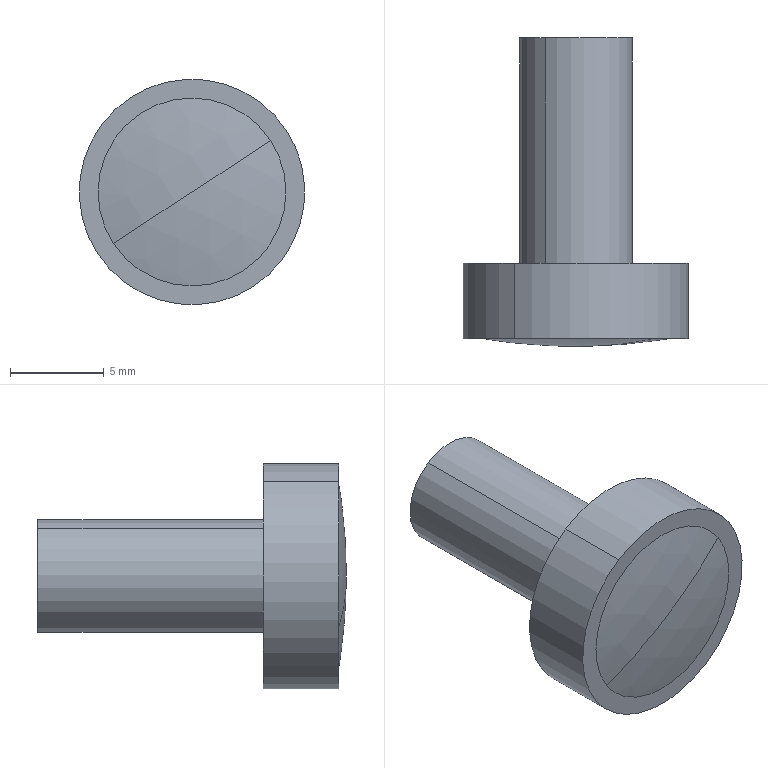Component | SolidWorks | SmallHandwheel-2 | 1 solid | 9 faces | box 12 x 16.42 x 12 mm | volume 808 mm3 | cylinder 4 | plane 3 | sphere 2 | commonest cylinder face diameters 6 x2 12 x2
STEP:
#1=CARTESIAN_POINT('',(7.97,20.827,-9.056));
#2=VERTEX_POINT('',#1);
#3=CARTESIAN_POINT('',(7.841,20.827,-8.858));
#4=VERTEX_POINT('',#3);
#5=CARTESIAN_POINT('',(7.905,20.827,-8.957));
#6=DIRECTION('',(0.,1.,-0.));
#7=DIRECTION('',(0.5469,0.,-0.8372));
#8=AXIS2_PLACEMENT_3D('',#5,#6,#7);
#9=CIRCLE('',#8,0.1181);
#10=EDGE_CURVE('',#2,#4,#9,.T.);
#11=ORIENTED_EDGE('',*,*,#10,.T.);
#12=CARTESIAN_POINT('',(7.841,21.299,-8.858));
#13=VERTEX_POINT('',#12);
#14=CARTESIAN_POINT('',(7.841,21.299,-8.858));
#15=DIRECTION('',(0.,1.,-0.));
#16=VECTOR('',#15,39.37);
#17=LINE('',#14,#16);
#18=EDGE_CURVE('',#4,#13,#17,.T.);
#19=ORIENTED_EDGE('',*,*,#18,.T.);
#20=CARTESIAN_POINT('',(7.97,21.299,-9.056));
#21=VERTEX_POINT('',#20);
#22=CARTESIAN_POINT('',(7.905,21.299,-8.957));
#23=DIRECTION('',(-0.,-1.,0.));
#24=DIRECTION('',(0.5469,0.,-0.8372));
#25=AXIS2_PLACEMENT_3D('',#22,#23,#24);
#26=CIRCLE('',#25,0.1181);
#27=EDGE_CURVE('',#13,#21,#26,.T.);
#28=ORIENTED_EDGE('',*,*,#27,.T.);
#29=CARTESIAN_POINT('',(7.97,21.299,-9.056));
#30=DIRECTION('',(0.,1.,-0.));
#31=VECTOR('',#30,39.37);
#32=LINE('',#29,#31);
#33=EDGE_CURVE('',#2,#21,#32,.T.);
#34=ORIENTED_EDGE('',*,*,#33,.F.);
#35=EDGE_LOOP('',(#11,#19,#28,#34));
#36=FACE_OUTER_BOUND('',#35,.T.);
#37=CARTESIAN_POINT('',(7.905,21.299,-8.957));
#38=DIRECTION('',(0.,1.,-0.));
#39=DIRECTION('',(0.5469,0.,-0.8372));
#40=AXIS2_PLACEMENT_3D('',#37,#38,#39);
#41=CYLINDRICAL_SURFACE('',#40,0.1181);
#42=ADVANCED_FACE('',(#36),#41,.T.);
#43=CARTESIAN_POINT('',(8.034,20.669,-9.154));
#44=VERTEX_POINT('',#43);
#45=CARTESIAN_POINT('',(7.776,20.669,-8.759));
#46=VERTEX_POINT('',#45);
#47=CARTESIAN_POINT('',(7.905,20.669,-8.957));
#48=DIRECTION('',(0.,1.,-0.));
#49=DIRECTION('',(0.5469,0.,-0.8372));
#50=AXIS2_PLACEMENT_3D('',#47,#48,#49);
#51=CIRCLE('',#50,0.2362);
#52=EDGE_CURVE('',#44,#46,#51,.T.);
#53=ORIENTED_EDGE('',*,*,#52,.T.);
#54=CARTESIAN_POINT('',(7.776,20.827,-8.759));
#55=VERTEX_POINT('',#54);
#56=CARTESIAN_POINT('',(7.776,21.299,-8.759));
#57=DIRECTION('',(0.,1.,-0.));
#58=VECTOR('',#57,39.37);
#59=LINE('',#56,#58);
#60=EDGE_CURVE('',#46,#55,#59,.T.);
#61=ORIENTED_EDGE('',*,*,#60,.T.);
#62=CARTESIAN_POINT('',(8.034,20.827,-9.154));
#63=VERTEX_POINT('',#62);
#64=CARTESIAN_POINT('',(7.905,20.827,-8.957));
#65=DIRECTION('',(-0.,-1.,0.));
#66=DIRECTION('',(0.5469,0.,-0.8372));
#67=AXIS2_PLACEMENT_3D('',#64,#65,#66);
#68=CIRCLE('',#67,0.2362);
#69=EDGE_CURVE('',#55,#63,#68,.T.);
#70=ORIENTED_EDGE('',*,*,#69,.T.);
#71=CARTESIAN_POINT('',(8.034,21.299,-9.154));
#72=DIRECTION('',(0.,1.,-0.));
#73=VECTOR('',#72,39.37);
#74=LINE('',#71,#73);
#75=EDGE_CURVE('',#44,#63,#74,.T.);
#76=ORIENTED_EDGE('',*,*,#75,.F.);
#77=EDGE_LOOP('',(#53,#61,#70,#76));
#78=FACE_OUTER_BOUND('',#77,.T.);
#79=CARTESIAN_POINT('',(7.905,21.299,-8.957));
#80=DIRECTION('',(0.,1.,-0.));
#81=DIRECTION('',(0.5469,0.,-0.8372));
#82=AXIS2_PLACEMENT_3D('',#79,#80,#81);
#83=CYLINDRICAL_SURFACE('',#82,0.2362);
#84=ADVANCED_FACE('',(#78),#83,.T.);
#85=CARTESIAN_POINT('',(8.07,20.669,-8.849));
#86=VERTEX_POINT('',#85);
#87=CARTESIAN_POINT('',(7.74,20.669,-9.064));
#88=VERTEX_POINT('',#87);
#89=CARTESIAN_POINT('',(7.905,20.669,-8.957));
#90=DIRECTION('',(-0.,-1.,0.));
#91=DIRECTION('',(0.5469,0.,-0.8372));
#92=AXIS2_PLACEMENT_3D('',#89,#90,#91);
#93=CIRCLE('',#92,0.1969);
#94=EDGE_CURVE('',#86,#88,#93,.T.);
#95=ORIENTED_EDGE('',*,*,#94,.T.);
#96=CARTESIAN_POINT('',(7.905,21.834,-8.957));
#97=DIRECTION('',(-0.5469,0.,0.8372));
#98=DIRECTION('',(0.8372,0.,0.5469));
#99=AXIS2_PLACEMENT_3D('',#96,#97,#98);
#100=CIRCLE('',#99,1.181);
#101=EDGE_CURVE('',#88,#86,#100,.T.);
#102=ORIENTED_EDGE('',*,*,#101,.T.);
#103=EDGE_LOOP('',(#95,#102));
#104=FACE_OUTER_BOUND('',#103,.T.);
#105=CARTESIAN_POINT('',(7.905,21.834,-8.957));
#106=DIRECTION('',(0.5469,0.,-0.8372));
#107=DIRECTION('',(0.,-1.,0.));
#108=AXIS2_PLACEMENT_3D('',#105,#106,#107);
#109=SPHERICAL_SURFACE('',#108,1.181);
#110=ADVANCED_FACE('',(#104),#109,.T.);
#111=ORIENTED_EDGE('',*,*,#18,.F.);
#112=CARTESIAN_POINT('',(7.905,20.827,-8.957));
#113=DIRECTION('',(0.,1.,-0.));
#114=DIRECTION('',(0.5469,0.,-0.8372));
#115=AXIS2_PLACEMENT_3D('',#112,#113,#114);
#116=CIRCLE('',#115,0.1181);
#117=EDGE_CURVE('',#4,#2,#116,.T.);
#118=ORIENTED_EDGE('',*,*,#117,.T.);
#119=ORIENTED_EDGE('',*,*,#33,.T.);
#120=CARTESIAN_POINT('',(7.905,21.299,-8.957));
#121=DIRECTION('',(-0.,-1.,0.));
#122=DIRECTION('',(0.5469,0.,-0.8372));
#123=AXIS2_PLACEMENT_3D('',#120,#121,#122);
#124=CIRCLE('',#123,0.1181);
#125=EDGE_CURVE('',#21,#13,#124,.T.);
#126=ORIENTED_EDGE('',*,*,#125,.T.);
#127=EDGE_LOOP('',(#111,#118,#119,#126));
#128=FACE_OUTER_BOUND('',#127,.T.);
#129=CARTESIAN_POINT('',(7.905,21.299,-8.957));
#130=DIRECTION('',(0.,1.,-0.));
#131=DIRECTION('',(0.5469,0.,-0.8372));
#132=AXIS2_PLACEMENT_3D('',#129,#130,#131);
#133=CYLINDRICAL_SURFACE('',#132,0.1181);
#134=ADVANCED_FACE('',(#128),#133,.T.);
#135=ORIENTED_EDGE('',*,*,#125,.F.);
#136=ORIENTED_EDGE('',*,*,#27,.F.);
#137=EDGE_LOOP('',(#135,#136));
#138=FACE_OUTER_BOUND('',#137,.T.);
#139=CARTESIAN_POINT('',(8.004,21.299,-8.892));
#140=DIRECTION('',(-0.,-1.,0.));
#141=DIRECTION('',(-0.5469,0.,0.8372));
#142=AXIS2_PLACEMENT_3D('',#139,#140,#141);
#143=PLANE('',#142);
#144=ADVANCED_FACE('',(#138),#143,.F.);
#145=ORIENTED_EDGE('',*,*,#10,.F.);
#146=ORIENTED_EDGE('',*,*,#117,.F.);
#147=EDGE_LOOP('',(#145,#146));
#148=FACE_BOUND('',#147,.T.);
#149=CARTESIAN_POINT('',(7.905,20.827,-8.957));
#150=DIRECTION('',(-0.,-1.,0.));
#151=DIRECTION('',(0.5469,0.,-0.8372));
#152=AXIS2_PLACEMENT_3D('',#149,#150,#151);
#153=CIRCLE('',#152,0.2362);
#154=EDGE_CURVE('',#63,#55,#153,.T.);
#155=ORIENTED_EDGE('',*,*,#154,.F.);
#156=ORIENTED_EDGE('',*,*,#69,.F.);
#157=EDGE_LOOP('',(#155,#156));
#158=FACE_OUTER_BOUND('',#157,.T.);
#159=CARTESIAN_POINT('',(8.103,20.827,-8.827));
#160=DIRECTION('',(-0.,-1.,0.));
#161=DIRECTION('',(-0.5469,0.,0.8372));
#162=AXIS2_PLACEMENT_3D('',#159,#160,#161);
#163=PLANE('',#162);
#164=ADVANCED_FACE('',(#148,#158),#163,.F.);
#165=ORIENTED_EDGE('',*,*,#60,.F.);
#166=CARTESIAN_POINT('',(7.905,20.669,-8.957));
#167=DIRECTION('',(0.,1.,-0.));
#168=DIRECTION('',(0.5469,0.,-0.8372));
#169=AXIS2_PLACEMENT_3D('',#166,#167,#168);
#170=CIRCLE('',#169,0.2362);
#171=EDGE_CURVE('',#46,#44,#170,.T.);
#172=ORIENTED_EDGE('',*,*,#171,.T.);
#173=ORIENTED_EDGE('',*,*,#75,.T.);
#174=ORIENTED_EDGE('',*,*,#154,.T.);
#175=EDGE_LOOP('',(#165,#172,#173,#174));
#176=FACE_OUTER_BOUND('',#175,.T.);
#177=CARTESIAN_POINT('',(7.905,21.299,-8.957));
#178=DIRECTION('',(0.,1.,-0.));
#179=DIRECTION('',(0.5469,0.,-0.8372));
#180=AXIS2_PLACEMENT_3D('',#177,#178,#179);
#181=CYLINDRICAL_SURFACE('',#180,0.2362);
#182=ADVANCED_FACE('',(#176),#181,.T.);
#183=ORIENTED_EDGE('',*,*,#52,.F.);
#184=ORIENTED_EDGE('',*,*,#171,.F.);
#185=EDGE_LOOP('',(#183,#184));
#186=FACE_OUTER_BOUND('',#185,.T.);
#187=ORIENTED_EDGE('',*,*,#94,.F.);
#188=CARTESIAN_POINT('',(7.905,20.669,-8.957));
#189=DIRECTION('',(-0.,-1.,0.));
#190=DIRECTION('',(0.5469,0.,-0.8372));
#191=AXIS2_PLACEMENT_3D('',#188,#189,#190);
#192=CIRCLE('',#191,0.1969);
#193=EDGE_CURVE('',#88,#86,#192,.T.);
#194=ORIENTED_EDGE('',*,*,#193,.F.);
#195=EDGE_LOOP('',(#187,#194));
#196=FACE_BOUND('',#195,.T.);
#197=CARTESIAN_POINT('',(8.07,20.669,-8.849));
#198=DIRECTION('',(0.,1.,-0.));
#199=DIRECTION('',(0.5469,-0.,-0.8372));
#200=AXIS2_PLACEMENT_3D('',#197,#198,#199);
#201=PLANE('',#200);
#202=ADVANCED_FACE('',(#186,#196),#201,.F.);
#203=ORIENTED_EDGE('',*,*,#101,.F.);
#204=ORIENTED_EDGE('',*,*,#193,.T.);
#205=EDGE_LOOP('',(#203,#204));
#206=FACE_OUTER_BOUND('',#205,.T.);
#207=CARTESIAN_POINT('',(7.905,21.834,-8.957));
#208=DIRECTION('',(0.5469,0.,-0.8372));
#209=DIRECTION('',(0.,-1.,0.));
#210=AXIS2_PLACEMENT_3D('',#207,#208,#209);
#211=SPHERICAL_SURFACE('',#210,1.181);
#212=ADVANCED_FACE('',(#206),#211,.T.);
#213=CLOSED_SHELL('',(#42,#84,#110,#134,#144,#164,#182,#202,#212));
#214=MANIFOLD_SOLID_BREP('',#213);
#215=CARTESIAN_POINT('',(0.,0.,0.));
#216=DIRECTION('',(0.,0.,1.));
#217=DIRECTION('',(1.,0.,0.));
#218=AXIS2_PLACEMENT_3D('',#215,#216,#217);
#219=(LENGTH_UNIT()NAMED_UNIT(*)SI_UNIT($,.METRE.));
#220=LENGTH_MEASURE_WITH_UNIT(LENGTH_MEASURE(0.0254),#219);
#221=DIMENSIONAL_EXPONENTS(1.,0.,0.,0.,0.,0.,0.);
#222=(CONVERSION_BASED_UNIT('',#220)LENGTH_UNIT()NAMED_UNIT(#221));
#223=UNCERTAINTY_MEASURE_WITH_UNIT(LENGTH_MEASURE(0.00001),#222,'','');
#224=(NAMED_UNIT(*)PLANE_ANGLE_UNIT()SI_UNIT($,.RADIAN.));
#225=(NAMED_UNIT(*)SI_UNIT($,.STERADIAN.)SOLID_ANGLE_UNIT());
#226=(GEOMETRIC_REPRESENTATION_CONTEXT(3)GLOBAL_UNCERTAINTY_ASSIGNED_CONTEXT((#223))GLOBAL_UNIT_ASSIGNED_CONTEXT((#222,#224,#225))REPRESENTATION_CONTEXT('',''));
#227=ADVANCED_BREP_SHAPE_REPRESENTATION('',(#214,#218),#226);
#228=COLOUR_RGB('',0.7922,0.8196,0.9333);
#229=FILL_AREA_STYLE_COLOUR('',#228);
#230=FILL_AREA_STYLE('',(#229));
#231=SURFACE_STYLE_FILL_AREA(#230);
#232=SURFACE_SIDE_STYLE('',(#231));
#233=SURFACE_STYLE_USAGE(.BOTH.,#232);
#234=PRESENTATION_STYLE_ASSIGNMENT((#233));
#235=STYLED_ITEM('',(#234),#214);
#236=(LENGTH_UNIT()NAMED_UNIT(*)SI_UNIT($,.METRE.));
#237=LENGTH_MEASURE_WITH_UNIT(LENGTH_MEASURE(0.0254),#236);
#238=DIMENSIONAL_EXPONENTS(1.,0.,0.,0.,0.,0.,0.);
#239=(CONVERSION_BASED_UNIT('',#237)LENGTH_UNIT()NAMED_UNIT(#238));
#240=UNCERTAINTY_MEASURE_WITH_UNIT(LENGTH_MEASURE(0.00001),#239,'','');
#241=(NAMED_UNIT(*)PLANE_ANGLE_UNIT()SI_UNIT($,.RADIAN.));
#242=(NAMED_UNIT(*)SI_UNIT($,.STERADIAN.)SOLID_ANGLE_UNIT());
#243=(GEOMETRIC_REPRESENTATION_CONTEXT(3)GLOBAL_UNCERTAINTY_ASSIGNED_CONTEXT((#240))GLOBAL_UNIT_ASSIGNED_CONTEXT((#239,#241,#242))REPRESENTATION_CONTEXT('',''));
#244=MECHANICAL_DESIGN_GEOMETRIC_PRESENTATION_REPRESENTATION('',(#235),#243);
#245=PRESENTATION_LAYER_ASSIGNMENT('','',(#235));